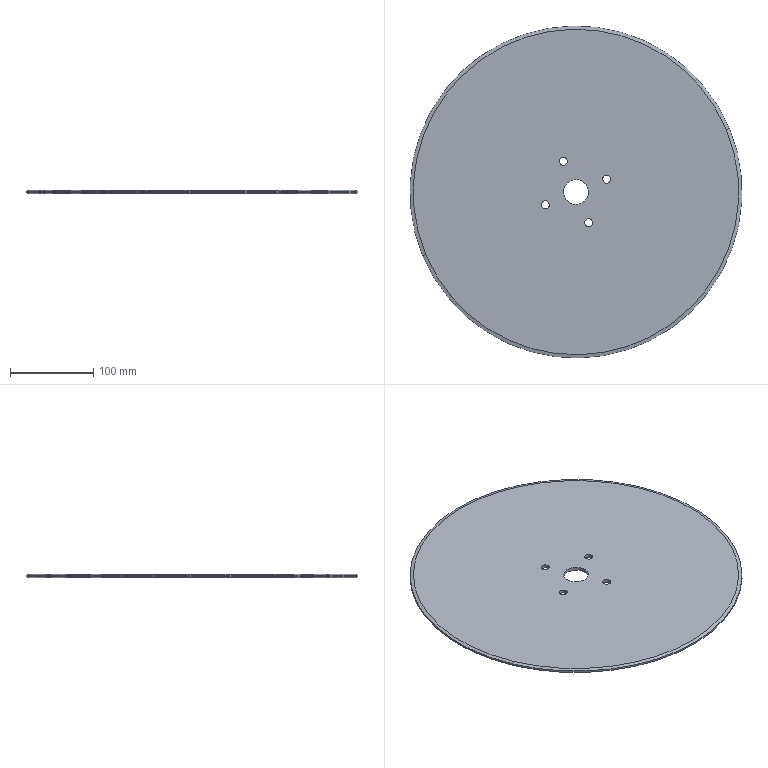Component | SolidWorks | SawBlade-1 | 1 solid | 18 faces | box 400 x 400 x 4.2 mm | volume 518276 mm3 | cylinder 12 | cone 4 | plane 2 | commonest cylinder face diameters 9.5 x8 30 x2 400 x2 | material 45
STEP:
#1=CARTESIAN_POINT('',(-21.82,48.885,7.508));
#2=VERTEX_POINT('',#1);
#3=CARTESIAN_POINT('',(-7.564,54.797,7.508));
#4=VERTEX_POINT('',#3);
#5=CARTESIAN_POINT('',(-14.692,51.841,7.508));
#6=DIRECTION('',(0.,0.,-1.));
#7=DIRECTION('',(0.9237,0.383,0.));
#8=AXIS2_PLACEMENT_3D('',#5,#6,#7);
#9=CIRCLE('',#8,7.717);
#10=EDGE_CURVE('',#2,#4,#9,.T.);
#11=ORIENTED_EDGE('',*,*,#10,.F.);
#12=CARTESIAN_POINT('',(-21.965,48.825,7.55));
#13=VERTEX_POINT('',#12);
#14=CARTESIAN_POINT('',(-21.965,48.825,7.55));
#15=DIRECTION('',(-0.8923,-0.37,0.2588));
#16=VECTOR('',#15,39.37);
#17=LINE('',#14,#16);
#18=EDGE_CURVE('',#2,#13,#17,.T.);
#19=ORIENTED_EDGE('',*,*,#18,.T.);
#20=CARTESIAN_POINT('',(-7.418,54.857,7.55));
#21=VERTEX_POINT('',#20);
#22=CARTESIAN_POINT('',(-14.692,51.841,7.55));
#23=DIRECTION('',(-0.,-0.,1.));
#24=DIRECTION('',(0.9237,0.383,0.));
#25=AXIS2_PLACEMENT_3D('',#22,#23,#24);
#26=CIRCLE('',#25,7.874);
#27=EDGE_CURVE('',#21,#13,#26,.T.);
#28=ORIENTED_EDGE('',*,*,#27,.F.);
#29=CARTESIAN_POINT('',(-7.418,54.857,7.55));
#30=DIRECTION('',(0.8923,0.37,0.2588));
#31=VECTOR('',#30,39.37);
#32=LINE('',#29,#31);
#33=EDGE_CURVE('',#4,#21,#32,.T.);
#34=ORIENTED_EDGE('',*,*,#33,.F.);
#35=EDGE_LOOP('',(#11,#19,#28,#34));
#36=FACE_OUTER_BOUND('',#35,.T.);
#37=CARTESIAN_POINT('',(-14.692,51.841,7.55));
#38=DIRECTION('',(-0.,-0.,1.));
#39=DIRECTION('',(0.9237,0.383,0.));
#40=AXIS2_PLACEMENT_3D('',#37,#38,#39);
#41=CONICAL_SURFACE('',#40,7.874,1.309);
#42=ADVANCED_FACE('',(#36),#41,.T.);
#43=CARTESIAN_POINT('',(-7.564,54.797,7.673));
#44=VERTEX_POINT('',#43);
#45=CARTESIAN_POINT('',(-21.82,48.885,7.673));
#46=VERTEX_POINT('',#45);
#47=CARTESIAN_POINT('',(-14.692,51.841,7.673));
#48=DIRECTION('',(-0.,-0.,1.));
#49=DIRECTION('',(0.9237,0.383,0.));
#50=AXIS2_PLACEMENT_3D('',#47,#48,#49);
#51=CIRCLE('',#50,7.717);
#52=EDGE_CURVE('',#44,#46,#51,.T.);
#53=ORIENTED_EDGE('',*,*,#52,.F.);
#54=CARTESIAN_POINT('',(-7.418,54.857,7.631));
#55=VERTEX_POINT('',#54);
#56=CARTESIAN_POINT('',(-7.564,54.797,7.673));
#57=DIRECTION('',(0.8923,0.37,-0.2588));
#58=VECTOR('',#57,39.37);
#59=LINE('',#56,#58);
#60=EDGE_CURVE('',#44,#55,#59,.T.);
#61=ORIENTED_EDGE('',*,*,#60,.T.);
#62=CARTESIAN_POINT('',(-21.965,48.825,7.631));
#63=VERTEX_POINT('',#62);
#64=CARTESIAN_POINT('',(-14.692,51.841,7.631));
#65=DIRECTION('',(0.,0.,-1.));
#66=DIRECTION('',(0.9237,0.383,0.));
#67=AXIS2_PLACEMENT_3D('',#64,#65,#66);
#68=CIRCLE('',#67,7.874);
#69=EDGE_CURVE('',#63,#55,#68,.T.);
#70=ORIENTED_EDGE('',*,*,#69,.F.);
#71=CARTESIAN_POINT('',(-21.82,48.885,7.673));
#72=DIRECTION('',(-0.8923,-0.37,-0.2588));
#73=VECTOR('',#72,39.37);
#74=LINE('',#71,#73);
#75=EDGE_CURVE('',#46,#63,#74,.T.);
#76=ORIENTED_EDGE('',*,*,#75,.F.);
#77=EDGE_LOOP('',(#53,#61,#70,#76));
#78=FACE_OUTER_BOUND('',#77,.T.);
#79=CARTESIAN_POINT('',(-14.692,51.841,7.673));
#80=DIRECTION('',(0.,0.,-1.));
#81=DIRECTION('',(-0.9237,-0.383,-0.));
#82=AXIS2_PLACEMENT_3D('',#79,#80,#81);
#83=CONICAL_SURFACE('',#82,7.717,1.309);
#84=ADVANCED_FACE('',(#78),#83,.T.);
#85=CARTESIAN_POINT('',(-15.974,51.309,7.508));
#86=VERTEX_POINT('',#85);
#87=CARTESIAN_POINT('',(-16.319,51.166,7.508));
#88=VERTEX_POINT('',#87);
#89=CARTESIAN_POINT('',(-16.146,51.238,7.508));
#90=DIRECTION('',(0.,0.,-1.));
#91=DIRECTION('',(0.9237,0.383,0.));
#92=AXIS2_PLACEMENT_3D('',#89,#90,#91);
#93=CIRCLE('',#92,0.187);
#94=EDGE_CURVE('',#86,#88,#93,.T.);
#95=ORIENTED_EDGE('',*,*,#94,.T.);
#96=CARTESIAN_POINT('',(-16.319,51.166,7.673));
#97=VERTEX_POINT('',#96);
#98=CARTESIAN_POINT('',(-16.319,51.166,7.508));
#99=DIRECTION('',(-0.,-0.,1.));
#100=VECTOR('',#99,39.37);
#101=LINE('',#98,#100);
#102=EDGE_CURVE('',#88,#97,#101,.T.);
#103=ORIENTED_EDGE('',*,*,#102,.T.);
#104=CARTESIAN_POINT('',(-15.974,51.309,7.673));
#105=VERTEX_POINT('',#104);
#106=CARTESIAN_POINT('',(-16.146,51.238,7.673));
#107=DIRECTION('',(-0.,-0.,1.));
#108=DIRECTION('',(-0.383,0.9237,-0.));
#109=AXIS2_PLACEMENT_3D('',#106,#107,#108);
#110=CIRCLE('',#109,0.187);
#111=EDGE_CURVE('',#97,#105,#110,.T.);
#112=ORIENTED_EDGE('',*,*,#111,.T.);
#113=CARTESIAN_POINT('',(-15.974,51.309,7.508));
#114=DIRECTION('',(-0.,-0.,1.));
#115=VECTOR('',#114,39.37);
#116=LINE('',#113,#115);
#117=EDGE_CURVE('',#86,#105,#116,.T.);
#118=ORIENTED_EDGE('',*,*,#117,.F.);
#119=EDGE_LOOP('',(#95,#103,#112,#118));
#120=FACE_OUTER_BOUND('',#119,.T.);
#121=CARTESIAN_POINT('',(-16.146,51.238,7.508));
#122=DIRECTION('',(-0.,-0.,1.));
#123=DIRECTION('',(0.9237,0.383,0.));
#124=AXIS2_PLACEMENT_3D('',#121,#122,#123);
#125=CYLINDRICAL_SURFACE('',#124,0.187);
#126=ADVANCED_FACE('',(#120),#125,.F.);
#127=CARTESIAN_POINT('',(-13.916,50.458,7.508));
#128=VERTEX_POINT('',#127);
#129=CARTESIAN_POINT('',(-14.261,50.315,7.508));
#130=VERTEX_POINT('',#129);
#131=CARTESIAN_POINT('',(-14.088,50.386,7.508));
#132=DIRECTION('',(0.,0.,-1.));
#133=DIRECTION('',(0.9237,0.383,0.));
#134=AXIS2_PLACEMENT_3D('',#131,#132,#133);
#135=CIRCLE('',#134,0.187);
#136=EDGE_CURVE('',#128,#130,#135,.T.);
#137=ORIENTED_EDGE('',*,*,#136,.T.);
#138=CARTESIAN_POINT('',(-14.261,50.315,7.673));
#139=VERTEX_POINT('',#138);
#140=CARTESIAN_POINT('',(-14.261,50.315,7.508));
#141=DIRECTION('',(-0.,-0.,1.));
#142=VECTOR('',#141,39.37);
#143=LINE('',#140,#142);
#144=EDGE_CURVE('',#130,#139,#143,.T.);
#145=ORIENTED_EDGE('',*,*,#144,.T.);
#146=CARTESIAN_POINT('',(-13.916,50.458,7.673));
#147=VERTEX_POINT('',#146);
#148=CARTESIAN_POINT('',(-14.088,50.386,7.673));
#149=DIRECTION('',(-0.,-0.,1.));
#150=DIRECTION('',(-0.9237,-0.383,-0.));
#151=AXIS2_PLACEMENT_3D('',#148,#149,#150);
#152=CIRCLE('',#151,0.187);
#153=EDGE_CURVE('',#139,#147,#152,.T.);
#154=ORIENTED_EDGE('',*,*,#153,.T.);
#155=CARTESIAN_POINT('',(-13.916,50.458,7.508));
#156=DIRECTION('',(-0.,-0.,1.));
#157=VECTOR('',#156,39.37);
#158=LINE('',#155,#157);
#159=EDGE_CURVE('',#128,#147,#158,.T.);
#160=ORIENTED_EDGE('',*,*,#159,.F.);
#161=EDGE_LOOP('',(#137,#145,#154,#160));
#162=FACE_OUTER_BOUND('',#161,.T.);
#163=CARTESIAN_POINT('',(-14.088,50.386,7.508));
#164=DIRECTION('',(-0.,-0.,1.));
#165=DIRECTION('',(0.9237,0.383,0.));
#166=AXIS2_PLACEMENT_3D('',#163,#164,#165);
#167=CYLINDRICAL_SURFACE('',#166,0.187);
#168=ADVANCED_FACE('',(#162),#167,.F.);
#169=CARTESIAN_POINT('',(-13.064,52.516,7.508));
#170=VERTEX_POINT('',#169);
#171=CARTESIAN_POINT('',(-13.41,52.373,7.508));
#172=VERTEX_POINT('',#171);
#173=CARTESIAN_POINT('',(-13.237,52.444,7.508));
#174=DIRECTION('',(0.,0.,-1.));
#175=DIRECTION('',(0.9237,0.383,0.));
#176=AXIS2_PLACEMENT_3D('',#173,#174,#175);
#177=CIRCLE('',#176,0.187);
#178=EDGE_CURVE('',#170,#172,#177,.T.);
#179=ORIENTED_EDGE('',*,*,#178,.T.);
#180=CARTESIAN_POINT('',(-13.41,52.373,7.673));
#181=VERTEX_POINT('',#180);
#182=CARTESIAN_POINT('',(-13.41,52.373,7.508));
#183=DIRECTION('',(-0.,-0.,1.));
#184=VECTOR('',#183,39.37);
#185=LINE('',#182,#184);
#186=EDGE_CURVE('',#172,#181,#185,.T.);
#187=ORIENTED_EDGE('',*,*,#186,.T.);
#188=CARTESIAN_POINT('',(-13.064,52.516,7.673));
#189=VERTEX_POINT('',#188);
#190=CARTESIAN_POINT('',(-13.237,52.444,7.673));
#191=DIRECTION('',(-0.,-0.,1.));
#192=DIRECTION('',(0.383,-0.9237,0.));
#193=AXIS2_PLACEMENT_3D('',#190,#191,#192);
#194=CIRCLE('',#193,0.187);
#195=EDGE_CURVE('',#181,#189,#194,.T.);
#196=ORIENTED_EDGE('',*,*,#195,.T.);
#197=CARTESIAN_POINT('',(-13.064,52.516,7.508));
#198=DIRECTION('',(-0.,-0.,1.));
#199=VECTOR('',#198,39.37);
#200=LINE('',#197,#199);
#201=EDGE_CURVE('',#170,#189,#200,.T.);
#202=ORIENTED_EDGE('',*,*,#201,.F.);
#203=EDGE_LOOP('',(#179,#187,#196,#202));
#204=FACE_OUTER_BOUND('',#203,.T.);
#205=CARTESIAN_POINT('',(-13.237,52.444,7.508));
#206=DIRECTION('',(-0.,-0.,1.));
#207=DIRECTION('',(0.9237,0.383,0.));
#208=AXIS2_PLACEMENT_3D('',#205,#206,#207);
#209=CYLINDRICAL_SURFACE('',#208,0.187);
#210=ADVANCED_FACE('',(#204),#209,.F.);
#211=CARTESIAN_POINT('',(-15.122,53.367,7.508));
#212=VERTEX_POINT('',#211);
#213=CARTESIAN_POINT('',(-15.468,53.224,7.508));
#214=VERTEX_POINT('',#213);
#215=CARTESIAN_POINT('',(-15.295,53.296,7.508));
#216=DIRECTION('',(0.,0.,-1.));
#217=DIRECTION('',(0.9237,0.383,0.));
#218=AXIS2_PLACEMENT_3D('',#215,#216,#217);
#219=CIRCLE('',#218,0.187);
#220=EDGE_CURVE('',#212,#214,#219,.T.);
#221=ORIENTED_EDGE('',*,*,#220,.T.);
#222=CARTESIAN_POINT('',(-15.468,53.224,7.673));
#223=VERTEX_POINT('',#222);
#224=CARTESIAN_POINT('',(-15.468,53.224,7.508));
#225=DIRECTION('',(-0.,-0.,1.));
#226=VECTOR('',#225,39.37);
#227=LINE('',#224,#226);
#228=EDGE_CURVE('',#214,#223,#227,.T.);
#229=ORIENTED_EDGE('',*,*,#228,.T.);
#230=CARTESIAN_POINT('',(-15.122,53.367,7.673));
#231=VERTEX_POINT('',#230);
#232=CARTESIAN_POINT('',(-15.295,53.296,7.673));
#233=DIRECTION('',(-0.,-0.,1.));
#234=DIRECTION('',(0.9237,0.383,0.));
#235=AXIS2_PLACEMENT_3D('',#232,#233,#234);
#236=CIRCLE('',#235,0.187);
#237=EDGE_CURVE('',#223,#231,#236,.T.);
#238=ORIENTED_EDGE('',*,*,#237,.T.);
#239=CARTESIAN_POINT('',(-15.122,53.367,7.508));
#240=DIRECTION('',(-0.,-0.,1.));
#241=VECTOR('',#240,39.37);
#242=LINE('',#239,#241);
#243=EDGE_CURVE('',#212,#231,#242,.T.);
#244=ORIENTED_EDGE('',*,*,#243,.F.);
#245=EDGE_LOOP('',(#221,#229,#238,#244));
#246=FACE_OUTER_BOUND('',#245,.T.);
#247=CARTESIAN_POINT('',(-15.295,53.296,7.508));
#248=DIRECTION('',(-0.,-0.,1.));
#249=DIRECTION('',(0.9237,0.383,0.));
#250=AXIS2_PLACEMENT_3D('',#247,#248,#249);
#251=CYLINDRICAL_SURFACE('',#250,0.187);
#252=ADVANCED_FACE('',(#246),#251,.F.);
#253=CARTESIAN_POINT('',(-15.237,51.615,7.673));
#254=VERTEX_POINT('',#253);
#255=CARTESIAN_POINT('',(-14.146,52.067,7.673));
#256=VERTEX_POINT('',#255);
#257=CARTESIAN_POINT('',(-14.692,51.841,7.673));
#258=DIRECTION('',(-0.,-0.,1.));
#259=DIRECTION('',(0.9237,0.383,0.));
#260=AXIS2_PLACEMENT_3D('',#257,#258,#259);
#261=CIRCLE('',#260,0.5906);
#262=EDGE_CURVE('',#254,#256,#261,.T.);
#263=ORIENTED_EDGE('',*,*,#262,.T.);
#264=CARTESIAN_POINT('',(-14.146,52.067,7.508));
#265=VERTEX_POINT('',#264);
#266=CARTESIAN_POINT('',(-14.146,52.067,7.673));
#267=DIRECTION('',(0.,0.,-1.));
#268=VECTOR('',#267,39.37);
#269=LINE('',#266,#268);
#270=EDGE_CURVE('',#256,#265,#269,.T.);
#271=ORIENTED_EDGE('',*,*,#270,.T.);
#272=CARTESIAN_POINT('',(-15.237,51.615,7.508));
#273=VERTEX_POINT('',#272);
#274=CARTESIAN_POINT('',(-14.692,51.841,7.508));
#275=DIRECTION('',(-0.,-0.,1.));
#276=DIRECTION('',(0.9237,0.383,0.));
#277=AXIS2_PLACEMENT_3D('',#274,#275,#276);
#278=CIRCLE('',#277,0.5906);
#279=EDGE_CURVE('',#273,#265,#278,.T.);
#280=ORIENTED_EDGE('',*,*,#279,.F.);
#281=CARTESIAN_POINT('',(-15.237,51.615,7.673));
#282=DIRECTION('',(0.,0.,-1.));
#283=VECTOR('',#282,39.37);
#284=LINE('',#281,#283);
#285=EDGE_CURVE('',#254,#273,#284,.T.);
#286=ORIENTED_EDGE('',*,*,#285,.F.);
#287=EDGE_LOOP('',(#263,#271,#280,#286));
#288=FACE_OUTER_BOUND('',#287,.T.);
#289=CARTESIAN_POINT('',(-14.692,51.841,7.673));
#290=DIRECTION('',(0.,0.,-1.));
#291=DIRECTION('',(-0.9237,-0.383,-0.));
#292=AXIS2_PLACEMENT_3D('',#289,#290,#291);
#293=CYLINDRICAL_SURFACE('',#292,0.5906);
#294=ADVANCED_FACE('',(#288),#293,.F.);
#295=ORIENTED_EDGE('',*,*,#69,.T.);
#296=CARTESIAN_POINT('',(-7.418,54.857,7.673));
#297=DIRECTION('',(0.,0.,-1.));
#298=VECTOR('',#297,39.37);
#299=LINE('',#296,#298);
#300=EDGE_CURVE('',#55,#21,#299,.T.);
#301=ORIENTED_EDGE('',*,*,#300,.T.);
#302=ORIENTED_EDGE('',*,*,#27,.T.);
#303=CARTESIAN_POINT('',(-21.965,48.825,7.673));
#304=DIRECTION('',(0.,0.,-1.));
#305=VECTOR('',#304,39.37);
#306=LINE('',#303,#305);
#307=EDGE_CURVE('',#63,#13,#306,.T.);
#308=ORIENTED_EDGE('',*,*,#307,.F.);
#309=EDGE_LOOP('',(#295,#301,#302,#308));
#310=FACE_OUTER_BOUND('',#309,.T.);
#311=CARTESIAN_POINT('',(-14.692,51.841,7.673));
#312=DIRECTION('',(0.,0.,-1.));
#313=DIRECTION('',(-0.9237,-0.383,-0.));
#314=AXIS2_PLACEMENT_3D('',#311,#312,#313);
#315=CYLINDRICAL_SURFACE('',#314,7.874);
#316=ADVANCED_FACE('',(#310),#315,.T.);
#317=CARTESIAN_POINT('',(-14.692,51.841,7.673));
#318=DIRECTION('',(-0.,-0.,1.));
#319=DIRECTION('',(0.9237,0.383,0.));
#320=AXIS2_PLACEMENT_3D('',#317,#318,#319);
#321=CIRCLE('',#320,7.717);
#322=EDGE_CURVE('',#46,#44,#321,.T.);
#323=ORIENTED_EDGE('',*,*,#322,.T.);
#324=ORIENTED_EDGE('',*,*,#52,.T.);
#325=EDGE_LOOP('',(#323,#324));
#326=FACE_OUTER_BOUND('',#325,.T.);
#327=CARTESIAN_POINT('',(-16.146,51.238,7.673));
#328=DIRECTION('',(-0.,-0.,1.));
#329=DIRECTION('',(-0.383,0.9237,-0.));
#330=AXIS2_PLACEMENT_3D('',#327,#328,#329);
#331=CIRCLE('',#330,0.187);
#332=EDGE_CURVE('',#105,#97,#331,.T.);
#333=ORIENTED_EDGE('',*,*,#332,.F.);
#334=ORIENTED_EDGE('',*,*,#111,.F.);
#335=EDGE_LOOP('',(#333,#334));
#336=FACE_BOUND('',#335,.T.);
#337=CARTESIAN_POINT('',(-14.088,50.386,7.673));
#338=DIRECTION('',(-0.,-0.,1.));
#339=DIRECTION('',(-0.9237,-0.383,-0.));
#340=AXIS2_PLACEMENT_3D('',#337,#338,#339);
#341=CIRCLE('',#340,0.187);
#342=EDGE_CURVE('',#147,#139,#341,.T.);
#343=ORIENTED_EDGE('',*,*,#342,.F.);
#344=ORIENTED_EDGE('',*,*,#153,.F.);
#345=EDGE_LOOP('',(#343,#344));
#346=FACE_BOUND('',#345,.T.);
#347=CARTESIAN_POINT('',(-13.237,52.444,7.673));
#348=DIRECTION('',(-0.,-0.,1.));
#349=DIRECTION('',(0.383,-0.9237,0.));
#350=AXIS2_PLACEMENT_3D('',#347,#348,#349);
#351=CIRCLE('',#350,0.187);
#352=EDGE_CURVE('',#189,#181,#351,.T.);
#353=ORIENTED_EDGE('',*,*,#352,.F.);
#354=ORIENTED_EDGE('',*,*,#195,.F.);
#355=EDGE_LOOP('',(#353,#354));
#356=FACE_BOUND('',#355,.T.);
#357=CARTESIAN_POINT('',(-15.295,53.296,7.673));
#358=DIRECTION('',(-0.,-0.,1.));
#359=DIRECTION('',(0.9237,0.383,0.));
#360=AXIS2_PLACEMENT_3D('',#357,#358,#359);
#361=CIRCLE('',#360,0.187);
#362=EDGE_CURVE('',#231,#223,#361,.T.);
#363=ORIENTED_EDGE('',*,*,#362,.F.);
#364=ORIENTED_EDGE('',*,*,#237,.F.);
#365=EDGE_LOOP('',(#363,#364));
#366=FACE_BOUND('',#365,.T.);
#367=ORIENTED_EDGE('',*,*,#262,.F.);
#368=CARTESIAN_POINT('',(-14.692,51.841,7.673));
#369=DIRECTION('',(-0.,-0.,1.));
#370=DIRECTION('',(0.9237,0.383,0.));
#371=AXIS2_PLACEMENT_3D('',#368,#369,#370);
#372=CIRCLE('',#371,0.5906);
#373=EDGE_CURVE('',#256,#254,#372,.T.);
#374=ORIENTED_EDGE('',*,*,#373,.F.);
#375=EDGE_LOOP('',(#367,#374));
#376=FACE_BOUND('',#375,.T.);
#377=CARTESIAN_POINT('',(-14.692,51.841,7.673));
#378=DIRECTION('',(-0.,-0.,1.));
#379=DIRECTION('',(0.9237,0.383,0.));
#380=AXIS2_PLACEMENT_3D('',#377,#378,#379);
#381=PLANE('',#380);
#382=ADVANCED_FACE('',(#326,#336,#346,#356,#366,#376),#381,.T.);
#383=CARTESIAN_POINT('',(-14.692,51.841,7.508));
#384=DIRECTION('',(0.,0.,-1.));
#385=DIRECTION('',(0.9237,0.383,0.));
#386=AXIS2_PLACEMENT_3D('',#383,#384,#385);
#387=CIRCLE('',#386,7.717);
#388=EDGE_CURVE('',#4,#2,#387,.T.);
#389=ORIENTED_EDGE('',*,*,#388,.T.);
#390=ORIENTED_EDGE('',*,*,#10,.T.);
#391=EDGE_LOOP('',(#389,#390));
#392=FACE_OUTER_BOUND('',#391,.T.);
#393=ORIENTED_EDGE('',*,*,#94,.F.);
#394=CARTESIAN_POINT('',(-16.146,51.238,7.508));
#395=DIRECTION('',(0.,0.,-1.));
#396=DIRECTION('',(0.9237,0.383,0.));
#397=AXIS2_PLACEMENT_3D('',#394,#395,#396);
#398=CIRCLE('',#397,0.187);
#399=EDGE_CURVE('',#88,#86,#398,.T.);
#400=ORIENTED_EDGE('',*,*,#399,.F.);
#401=EDGE_LOOP('',(#393,#400));
#402=FACE_BOUND('',#401,.T.);
#403=ORIENTED_EDGE('',*,*,#136,.F.);
#404=CARTESIAN_POINT('',(-14.088,50.386,7.508));
#405=DIRECTION('',(0.,0.,-1.));
#406=DIRECTION('',(0.9237,0.383,0.));
#407=AXIS2_PLACEMENT_3D('',#404,#405,#406);
#408=CIRCLE('',#407,0.187);
#409=EDGE_CURVE('',#130,#128,#408,.T.);
#410=ORIENTED_EDGE('',*,*,#409,.F.);
#411=EDGE_LOOP('',(#403,#410));
#412=FACE_BOUND('',#411,.T.);
#413=ORIENTED_EDGE('',*,*,#178,.F.);
#414=CARTESIAN_POINT('',(-13.237,52.444,7.508));
#415=DIRECTION('',(0.,0.,-1.));
#416=DIRECTION('',(0.9237,0.383,0.));
#417=AXIS2_PLACEMENT_3D('',#414,#415,#416);
#418=CIRCLE('',#417,0.187);
#419=EDGE_CURVE('',#172,#170,#418,.T.);
#420=ORIENTED_EDGE('',*,*,#419,.F.);
#421=EDGE_LOOP('',(#413,#420));
#422=FACE_BOUND('',#421,.T.);
#423=ORIENTED_EDGE('',*,*,#220,.F.);
#424=CARTESIAN_POINT('',(-15.295,53.296,7.508));
#425=DIRECTION('',(0.,0.,-1.));
#426=DIRECTION('',(0.9237,0.383,0.));
#427=AXIS2_PLACEMENT_3D('',#424,#425,#426);
#428=CIRCLE('',#427,0.187);
#429=EDGE_CURVE('',#214,#212,#428,.T.);
#430=ORIENTED_EDGE('',*,*,#429,.F.);
#431=EDGE_LOOP('',(#423,#430));
#432=FACE_BOUND('',#431,.T.);
#433=ORIENTED_EDGE('',*,*,#279,.T.);
#434=CARTESIAN_POINT('',(-14.692,51.841,7.508));
#435=DIRECTION('',(-0.,-0.,1.));
#436=DIRECTION('',(0.9237,0.383,0.));
#437=AXIS2_PLACEMENT_3D('',#434,#435,#436);
#438=CIRCLE('',#437,0.5906);
#439=EDGE_CURVE('',#265,#273,#438,.T.);
#440=ORIENTED_EDGE('',*,*,#439,.T.);
#441=EDGE_LOOP('',(#433,#440));
#442=FACE_BOUND('',#441,.T.);
#443=CARTESIAN_POINT('',(-14.692,51.841,7.508));
#444=DIRECTION('',(-0.,-0.,1.));
#445=DIRECTION('',(0.9237,0.383,0.));
#446=AXIS2_PLACEMENT_3D('',#443,#444,#445);
#447=PLANE('',#446);
#448=ADVANCED_FACE('',(#392,#402,#412,#422,#432,#442),#447,.F.);
#449=ORIENTED_EDGE('',*,*,#300,.F.);
#450=CARTESIAN_POINT('',(-14.692,51.841,7.631));
#451=DIRECTION('',(0.,0.,-1.));
#452=DIRECTION('',(0.9237,0.383,0.));
#453=AXIS2_PLACEMENT_3D('',#450,#451,#452);
#454=CIRCLE('',#453,7.874);
#455=EDGE_CURVE('',#55,#63,#454,.T.);
#456=ORIENTED_EDGE('',*,*,#455,.T.);
#457=ORIENTED_EDGE('',*,*,#307,.T.);
#458=CARTESIAN_POINT('',(-14.692,51.841,7.55));
#459=DIRECTION('',(-0.,-0.,1.));
#460=DIRECTION('',(0.9237,0.383,0.));
#461=AXIS2_PLACEMENT_3D('',#458,#459,#460);
#462=CIRCLE('',#461,7.874);
#463=EDGE_CURVE('',#13,#21,#462,.T.);
#464=ORIENTED_EDGE('',*,*,#463,.T.);
#465=EDGE_LOOP('',(#449,#456,#457,#464));
#466=FACE_OUTER_BOUND('',#465,.T.);
#467=CARTESIAN_POINT('',(-14.692,51.841,7.673));
#468=DIRECTION('',(0.,0.,-1.));
#469=DIRECTION('',(-0.9237,-0.383,-0.));
#470=AXIS2_PLACEMENT_3D('',#467,#468,#469);
#471=CYLINDRICAL_SURFACE('',#470,7.874);
#472=ADVANCED_FACE('',(#466),#471,.T.);
#473=ORIENTED_EDGE('',*,*,#270,.F.);
#474=ORIENTED_EDGE('',*,*,#373,.T.);
#475=ORIENTED_EDGE('',*,*,#285,.T.);
#476=ORIENTED_EDGE('',*,*,#439,.F.);
#477=EDGE_LOOP('',(#473,#474,#475,#476));
#478=FACE_OUTER_BOUND('',#477,.T.);
#479=CARTESIAN_POINT('',(-14.692,51.841,7.673));
#480=DIRECTION('',(0.,0.,-1.));
#481=DIRECTION('',(-0.9237,-0.383,-0.));
#482=AXIS2_PLACEMENT_3D('',#479,#480,#481);
#483=CYLINDRICAL_SURFACE('',#482,0.5906);
#484=ADVANCED_FACE('',(#478),#483,.F.);
#485=ORIENTED_EDGE('',*,*,#228,.F.);
#486=ORIENTED_EDGE('',*,*,#429,.T.);
#487=ORIENTED_EDGE('',*,*,#243,.T.);
#488=ORIENTED_EDGE('',*,*,#362,.T.);
#489=EDGE_LOOP('',(#485,#486,#487,#488));
#490=FACE_OUTER_BOUND('',#489,.T.);
#491=CARTESIAN_POINT('',(-15.295,53.296,7.508));
#492=DIRECTION('',(-0.,-0.,1.));
#493=DIRECTION('',(0.9237,0.383,0.));
#494=AXIS2_PLACEMENT_3D('',#491,#492,#493);
#495=CYLINDRICAL_SURFACE('',#494,0.187);
#496=ADVANCED_FACE('',(#490),#495,.F.);
#497=ORIENTED_EDGE('',*,*,#186,.F.);
#498=ORIENTED_EDGE('',*,*,#419,.T.);
#499=ORIENTED_EDGE('',*,*,#201,.T.);
#500=ORIENTED_EDGE('',*,*,#352,.T.);
#501=EDGE_LOOP('',(#497,#498,#499,#500));
#502=FACE_OUTER_BOUND('',#501,.T.);
#503=CARTESIAN_POINT('',(-13.237,52.444,7.508));
#504=DIRECTION('',(-0.,-0.,1.));
#505=DIRECTION('',(0.9237,0.383,0.));
#506=AXIS2_PLACEMENT_3D('',#503,#504,#505);
#507=CYLINDRICAL_SURFACE('',#506,0.187);
#508=ADVANCED_FACE('',(#502),#507,.F.);
#509=ORIENTED_EDGE('',*,*,#144,.F.);
#510=ORIENTED_EDGE('',*,*,#409,.T.);
#511=ORIENTED_EDGE('',*,*,#159,.T.);
#512=ORIENTED_EDGE('',*,*,#342,.T.);
#513=EDGE_LOOP('',(#509,#510,#511,#512));
#514=FACE_OUTER_BOUND('',#513,.T.);
#515=CARTESIAN_POINT('',(-14.088,50.386,7.508));
#516=DIRECTION('',(-0.,-0.,1.));
#517=DIRECTION('',(0.9237,0.383,0.));
#518=AXIS2_PLACEMENT_3D('',#515,#516,#517);
#519=CYLINDRICAL_SURFACE('',#518,0.187);
#520=ADVANCED_FACE('',(#514),#519,.F.);
#521=ORIENTED_EDGE('',*,*,#102,.F.);
#522=ORIENTED_EDGE('',*,*,#399,.T.);
#523=ORIENTED_EDGE('',*,*,#117,.T.);
#524=ORIENTED_EDGE('',*,*,#332,.T.);
#525=EDGE_LOOP('',(#521,#522,#523,#524));
#526=FACE_OUTER_BOUND('',#525,.T.);
#527=CARTESIAN_POINT('',(-16.146,51.238,7.508));
#528=DIRECTION('',(-0.,-0.,1.));
#529=DIRECTION('',(0.9237,0.383,0.));
#530=AXIS2_PLACEMENT_3D('',#527,#528,#529);
#531=CYLINDRICAL_SURFACE('',#530,0.187);
#532=ADVANCED_FACE('',(#526),#531,.F.);
#533=ORIENTED_EDGE('',*,*,#60,.F.);
#534=ORIENTED_EDGE('',*,*,#322,.F.);
#535=ORIENTED_EDGE('',*,*,#75,.T.);
#536=ORIENTED_EDGE('',*,*,#455,.F.);
#537=EDGE_LOOP('',(#533,#534,#535,#536));
#538=FACE_OUTER_BOUND('',#537,.T.);
#539=CARTESIAN_POINT('',(-14.692,51.841,7.673));
#540=DIRECTION('',(0.,0.,-1.));
#541=DIRECTION('',(-0.9237,-0.383,-0.));
#542=AXIS2_PLACEMENT_3D('',#539,#540,#541);
#543=CONICAL_SURFACE('',#542,7.717,1.309);
#544=ADVANCED_FACE('',(#538),#543,.T.);
#545=ORIENTED_EDGE('',*,*,#18,.F.);
#546=ORIENTED_EDGE('',*,*,#388,.F.);
#547=ORIENTED_EDGE('',*,*,#33,.T.);
#548=ORIENTED_EDGE('',*,*,#463,.F.);
#549=EDGE_LOOP('',(#545,#546,#547,#548));
#550=FACE_OUTER_BOUND('',#549,.T.);
#551=CARTESIAN_POINT('',(-14.692,51.841,7.55));
#552=DIRECTION('',(-0.,-0.,1.));
#553=DIRECTION('',(0.9237,0.383,0.));
#554=AXIS2_PLACEMENT_3D('',#551,#552,#553);
#555=CONICAL_SURFACE('',#554,7.874,1.309);
#556=ADVANCED_FACE('',(#550),#555,.T.);
#557=CLOSED_SHELL('',(#42,#84,#126,#168,#210,#252,#294,#316,#382,#448,#472,#484,#496,#508,#520,#532,#544,#556));
#558=MANIFOLD_SOLID_BREP('',#557);
#559=CARTESIAN_POINT('',(0.,0.,0.));
#560=DIRECTION('',(0.,0.,1.));
#561=DIRECTION('',(1.,0.,0.));
#562=AXIS2_PLACEMENT_3D('',#559,#560,#561);
#563=(LENGTH_UNIT()NAMED_UNIT(*)SI_UNIT($,.METRE.));
#564=LENGTH_MEASURE_WITH_UNIT(LENGTH_MEASURE(0.0254),#563);
#565=DIMENSIONAL_EXPONENTS(1.,0.,0.,0.,0.,0.,0.);
#566=(CONVERSION_BASED_UNIT('',#564)LENGTH_UNIT()NAMED_UNIT(#565));
#567=UNCERTAINTY_MEASURE_WITH_UNIT(LENGTH_MEASURE(0.00001),#566,'','');
#568=(NAMED_UNIT(*)PLANE_ANGLE_UNIT()SI_UNIT($,.RADIAN.));
#569=(NAMED_UNIT(*)SI_UNIT($,.STERADIAN.)SOLID_ANGLE_UNIT());
#570=(GEOMETRIC_REPRESENTATION_CONTEXT(3)GLOBAL_UNCERTAINTY_ASSIGNED_CONTEXT((#567))GLOBAL_UNIT_ASSIGNED_CONTEXT((#566,#568,#569))REPRESENTATION_CONTEXT('',''));
#571=ADVANCED_BREP_SHAPE_REPRESENTATION('',(#558,#562),#570);
#572=COLOUR_RGB('',0.7922,0.8196,0.9333);
#573=FILL_AREA_STYLE_COLOUR('',#572);
#574=FILL_AREA_STYLE('',(#573));
#575=SURFACE_STYLE_FILL_AREA(#574);
#576=SURFACE_SIDE_STYLE('',(#575));
#577=SURFACE_STYLE_USAGE(.BOTH.,#576);
#578=PRESENTATION_STYLE_ASSIGNMENT((#577));
#579=STYLED_ITEM('',(#578),#558);
#580=PRESENTATION_LAYER_ASSIGNMENT('','',(#579));
#581=(LENGTH_UNIT()NAMED_UNIT(*)SI_UNIT($,.METRE.));
#582=LENGTH_MEASURE_WITH_UNIT(LENGTH_MEASURE(0.0254),#581);
#583=DIMENSIONAL_EXPONENTS(1.,0.,0.,0.,0.,0.,0.);
#584=(CONVERSION_BASED_UNIT('',#582)LENGTH_UNIT()NAMED_UNIT(#583));
#585=UNCERTAINTY_MEASURE_WITH_UNIT(LENGTH_MEASURE(0.00001),#584,'','');
#586=(NAMED_UNIT(*)PLANE_ANGLE_UNIT()SI_UNIT($,.RADIAN.));
#587=(NAMED_UNIT(*)SI_UNIT($,.STERADIAN.)SOLID_ANGLE_UNIT());
#588=(GEOMETRIC_REPRESENTATION_CONTEXT(3)GLOBAL_UNCERTAINTY_ASSIGNED_CONTEXT((#585))GLOBAL_UNIT_ASSIGNED_CONTEXT((#584,#586,#587))REPRESENTATION_CONTEXT('',''));
#589=MECHANICAL_DESIGN_GEOMETRIC_PRESENTATION_REPRESENTATION('',(#579),#588);